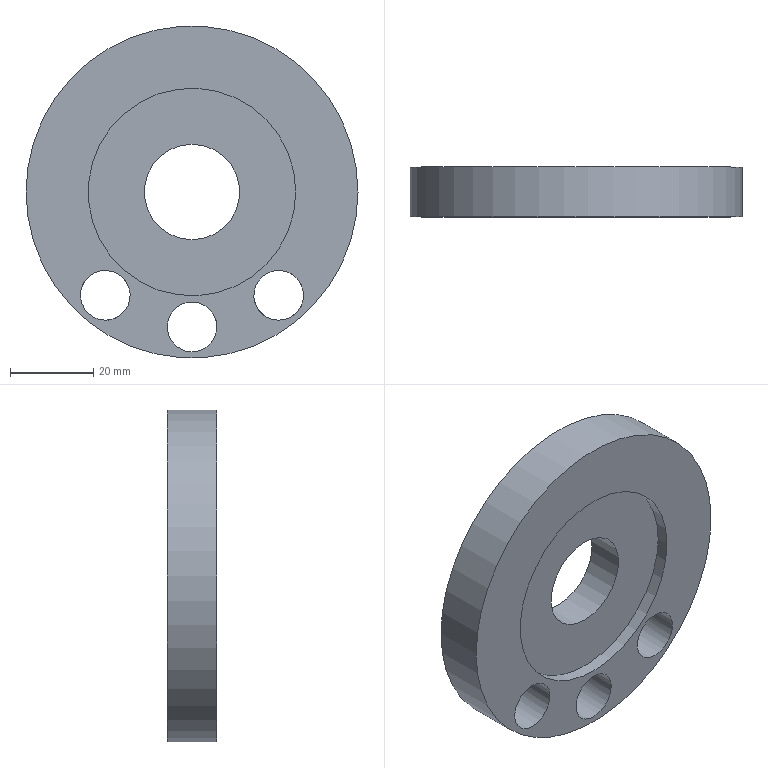Component | NX | INDEXING_PLATE | 1 solid | 9 faces | box 80 x 12 x 80 mm | volume 46617 mm3 | cylinder 6 | plane 3 | commonest cylinder face diameters 12 x3 80 x1 50 x1 23 x1
STEP:
#1=CARTESIAN_POINT('',(0.,0.,0.));
#2=DIRECTION('',(0.,0.,1.));
#3=DIRECTION('',(1.,0.,0.));
#4=AXIS2_PLACEMENT_3D('',#1,#2,#3);
#5=CARTESIAN_POINT('',(40.,-12.,66.));
#6=VERTEX_POINT('',#5);
#7=CARTESIAN_POINT('',(0.,-12.,66.));
#8=DIRECTION('',(0.,-1.,0.));
#9=DIRECTION('',(1.,0.,0.));
#10=AXIS2_PLACEMENT_3D('',#7,#8,#9);
#11=CIRCLE('',#10,40.);
#12=CARTESIAN_POINT('',(0.,-12.,66.));
#13=DIRECTION('',(0.,1.,0.));
#14=DIRECTION('',(0.,0.,1.));
#15=AXIS2_PLACEMENT_3D('',#12,#13,#14);
#16=CYLINDRICAL_SURFACE('',#15,40.);
#17=CARTESIAN_POINT('',(7.854,0.));
#18=DIRECTION('',(-1.,0.));
#19=VECTOR('',#18,1.);
#20=LINE('',#17,#19);
#21=(GEOMETRIC_REPRESENTATION_CONTEXT(2)PARAMETRIC_REPRESENTATION_CONTEXT()REPRESENTATION_CONTEXT('',''));
#22=DEFINITIONAL_REPRESENTATION('',(#20),#21);
#23=PCURVE('',#16,#22);
#24=CARTESIAN_POINT('',(0.,-12.,66.));
#25=DIRECTION('',(0.,-1.,0.));
#26=DIRECTION('',(0.,0.,-1.));
#27=AXIS2_PLACEMENT_3D('',#24,#25,#26);
#28=PLANE('',#27);
#29=CARTESIAN_POINT('',(0.,0.));
#30=DIRECTION('',(0.,1.));
#31=AXIS2_PLACEMENT_2D('',#29,#30);
#32=CIRCLE('',#31,40.);
#33=(GEOMETRIC_REPRESENTATION_CONTEXT(2)PARAMETRIC_REPRESENTATION_CONTEXT()REPRESENTATION_CONTEXT('',''));
#34=DEFINITIONAL_REPRESENTATION('',(#32),#33);
#35=PCURVE('',#28,#34);
#36=SURFACE_CURVE('',#11,(#23,#35),.PCURVE_S1.);
#37=EDGE_CURVE('',#6,#6,#36,.T.);
#38=ORIENTED_EDGE('',*,*,#37,.F.);
#39=CARTESIAN_POINT('',(40.,0.,66.));
#40=VERTEX_POINT('',#39);
#41=CARTESIAN_POINT('',(40.,-12.,66.));
#42=CARTESIAN_POINT('',(40.,0.,66.));
#43=B_SPLINE_CURVE_WITH_KNOTS('',1,(#41,#42),.UNSPECIFIED.,.F.,.F.,(2,2),(0.,12.),.PIECEWISE_BEZIER_KNOTS.);
#44=CARTESIAN_POINT('',(7.854,0.));
#45=DIRECTION('',(0.,1.));
#46=VECTOR('',#45,1.);
#47=LINE('',#44,#46);
#48=(GEOMETRIC_REPRESENTATION_CONTEXT(2)PARAMETRIC_REPRESENTATION_CONTEXT()REPRESENTATION_CONTEXT('',''));
#49=DEFINITIONAL_REPRESENTATION('',(#47),#48);
#50=PCURVE('',#16,#49);
#51=CARTESIAN_POINT('',(1.571,0.));
#52=DIRECTION('',(0.,1.));
#53=VECTOR('',#52,1.);
#54=LINE('',#51,#53);
#55=(GEOMETRIC_REPRESENTATION_CONTEXT(2)PARAMETRIC_REPRESENTATION_CONTEXT()REPRESENTATION_CONTEXT('',''));
#56=DEFINITIONAL_REPRESENTATION('',(#54),#55);
#57=PCURVE('',#16,#56);
#58=SEAM_CURVE('',#43,(#50,#57),.PCURVE_S1.);
#59=EDGE_CURVE('',#6,#40,#58,.T.);
#60=ORIENTED_EDGE('',*,*,#59,.T.);
#61=CARTESIAN_POINT('',(0.,0.,66.));
#62=DIRECTION('',(0.,-1.,0.));
#63=DIRECTION('',(1.,0.,0.));
#64=AXIS2_PLACEMENT_3D('',#61,#62,#63);
#65=CIRCLE('',#64,40.);
#66=CARTESIAN_POINT('',(7.854,12.));
#67=DIRECTION('',(-1.,0.));
#68=VECTOR('',#67,1.);
#69=LINE('',#66,#68);
#70=(GEOMETRIC_REPRESENTATION_CONTEXT(2)PARAMETRIC_REPRESENTATION_CONTEXT()REPRESENTATION_CONTEXT('',''));
#71=DEFINITIONAL_REPRESENTATION('',(#69),#70);
#72=PCURVE('',#16,#71);
#73=CARTESIAN_POINT('',(0.,0.,66.));
#74=DIRECTION('',(0.,-1.,0.));
#75=DIRECTION('',(0.,0.,-1.));
#76=AXIS2_PLACEMENT_3D('',#73,#74,#75);
#77=PLANE('',#76);
#78=CARTESIAN_POINT('',(0.,0.));
#79=DIRECTION('',(0.,1.));
#80=AXIS2_PLACEMENT_2D('',#78,#79);
#81=CIRCLE('',#80,40.);
#82=(GEOMETRIC_REPRESENTATION_CONTEXT(2)PARAMETRIC_REPRESENTATION_CONTEXT()REPRESENTATION_CONTEXT('',''));
#83=DEFINITIONAL_REPRESENTATION('',(#81),#82);
#84=PCURVE('',#77,#83);
#85=SURFACE_CURVE('',#65,(#72,#84),.PCURVE_S1.);
#86=EDGE_CURVE('',#40,#40,#85,.T.);
#87=ORIENTED_EDGE('',*,*,#86,.T.);
#88=ORIENTED_EDGE('',*,*,#59,.F.);
#89=EDGE_LOOP('',(#38,#60,#87,#88));
#90=FACE_BOUND('',#89,.T.);
#91=ADVANCED_FACE('',(#90),#16,.T.);
#92=CARTESIAN_POINT('',(26.891,-12.,41.104));
#93=VERTEX_POINT('',#92);
#94=CARTESIAN_POINT('',(20.891,-12.,35.104));
#95=VERTEX_POINT('',#94);
#96=CARTESIAN_POINT('',(20.891,-12.,41.104));
#97=DIRECTION('',(0.,-1.,0.));
#98=DIRECTION('',(1.,0.,0.));
#99=AXIS2_PLACEMENT_3D('',#96,#97,#98);
#100=CIRCLE('',#99,6.);
#101=CARTESIAN_POINT('',(24.896,20.891));
#102=DIRECTION('',(0.,1.));
#103=AXIS2_PLACEMENT_2D('',#101,#102);
#104=CIRCLE('',#103,6.);
#105=(GEOMETRIC_REPRESENTATION_CONTEXT(2)PARAMETRIC_REPRESENTATION_CONTEXT()REPRESENTATION_CONTEXT('',''));
#106=DEFINITIONAL_REPRESENTATION('',(#104),#105);
#107=PCURVE('',#28,#106);
#108=CARTESIAN_POINT('',(20.891,38.,41.104));
#109=DIRECTION('',(0.,-1.,0.));
#110=DIRECTION('',(0.,0.,-1.));
#111=AXIS2_PLACEMENT_3D('',#108,#109,#110);
#112=CYLINDRICAL_SURFACE('',#111,6.);
#113=CARTESIAN_POINT('',(1.571,50.));
#114=DIRECTION('',(1.,0.));
#115=VECTOR('',#114,1.);
#116=LINE('',#113,#115);
#117=(GEOMETRIC_REPRESENTATION_CONTEXT(2)PARAMETRIC_REPRESENTATION_CONTEXT()REPRESENTATION_CONTEXT('',''));
#118=DEFINITIONAL_REPRESENTATION('',(#116),#117);
#119=PCURVE('',#112,#118);
#120=SURFACE_CURVE('',#100,(#107,#119),.PCURVE_S1.);
#121=EDGE_CURVE('',#93,#95,#120,.T.);
#122=ORIENTED_EDGE('',*,*,#121,.F.);
#123=CARTESIAN_POINT('',(20.891,-12.,41.104));
#124=DIRECTION('',(0.,-1.,0.));
#125=DIRECTION('',(1.,0.,0.));
#126=AXIS2_PLACEMENT_3D('',#123,#124,#125);
#127=CIRCLE('',#126,6.);
#128=CARTESIAN_POINT('',(24.896,20.891));
#129=DIRECTION('',(0.,1.));
#130=AXIS2_PLACEMENT_2D('',#128,#129);
#131=CIRCLE('',#130,6.);
#132=(GEOMETRIC_REPRESENTATION_CONTEXT(2)PARAMETRIC_REPRESENTATION_CONTEXT()REPRESENTATION_CONTEXT('',''));
#133=DEFINITIONAL_REPRESENTATION('',(#131),#132);
#134=PCURVE('',#28,#133);
#135=CARTESIAN_POINT('',(-4.712,50.));
#136=DIRECTION('',(1.,0.));
#137=VECTOR('',#136,1.);
#138=LINE('',#135,#137);
#139=(GEOMETRIC_REPRESENTATION_CONTEXT(2)PARAMETRIC_REPRESENTATION_CONTEXT()REPRESENTATION_CONTEXT('',''));
#140=DEFINITIONAL_REPRESENTATION('',(#138),#139);
#141=PCURVE('',#112,#140);
#142=SURFACE_CURVE('',#127,(#134,#141),.PCURVE_S1.);
#143=EDGE_CURVE('',#95,#93,#142,.T.);
#144=ORIENTED_EDGE('',*,*,#143,.F.);
#145=EDGE_LOOP('',(#122,#144));
#146=FACE_BOUND('',#145,.T.);
#147=CARTESIAN_POINT('',(-19.849,-12.,35.195));
#148=VERTEX_POINT('',#147);
#149=CARTESIAN_POINT('',(-20.891,-12.,35.104));
#150=VERTEX_POINT('',#149);
#151=CARTESIAN_POINT('',(-20.891,-12.,41.104));
#152=DIRECTION('',(0.,-1.,0.));
#153=DIRECTION('',(0.1736,0.,-0.9848));
#154=AXIS2_PLACEMENT_3D('',#151,#152,#153);
#155=CIRCLE('',#154,6.);
#156=CARTESIAN_POINT('',(24.896,-20.891));
#157=DIRECTION('',(0.9848,0.1736));
#158=AXIS2_PLACEMENT_2D('',#156,#157);
#159=CIRCLE('',#158,6.);
#160=(GEOMETRIC_REPRESENTATION_CONTEXT(2)PARAMETRIC_REPRESENTATION_CONTEXT()REPRESENTATION_CONTEXT('',''));
#161=DEFINITIONAL_REPRESENTATION('',(#159),#160);
#162=PCURVE('',#28,#161);
#163=CARTESIAN_POINT('',(-20.891,38.,41.104));
#164=DIRECTION('',(0.,-1.,0.));
#165=DIRECTION('',(0.,0.,-1.));
#166=AXIS2_PLACEMENT_3D('',#163,#164,#165);
#167=CYLINDRICAL_SURFACE('',#166,6.);
#168=CARTESIAN_POINT('',(0.1745,50.));
#169=DIRECTION('',(1.,0.));
#170=VECTOR('',#169,1.);
#171=LINE('',#168,#170);
#172=(GEOMETRIC_REPRESENTATION_CONTEXT(2)PARAMETRIC_REPRESENTATION_CONTEXT()REPRESENTATION_CONTEXT('',''));
#173=DEFINITIONAL_REPRESENTATION('',(#171),#172);
#174=PCURVE('',#167,#173);
#175=SURFACE_CURVE('',#155,(#162,#174),.PCURVE_S1.);
#176=EDGE_CURVE('',#148,#150,#175,.T.);
#177=ORIENTED_EDGE('',*,*,#176,.F.);
#178=CARTESIAN_POINT('',(-20.891,-12.,41.104));
#179=DIRECTION('',(0.,-1.,0.));
#180=DIRECTION('',(0.1736,0.,-0.9848));
#181=AXIS2_PLACEMENT_3D('',#178,#179,#180);
#182=CIRCLE('',#181,6.);
#183=CARTESIAN_POINT('',(24.896,-20.891));
#184=DIRECTION('',(0.9848,0.1736));
#185=AXIS2_PLACEMENT_2D('',#183,#184);
#186=CIRCLE('',#185,6.);
#187=(GEOMETRIC_REPRESENTATION_CONTEXT(2)PARAMETRIC_REPRESENTATION_CONTEXT()REPRESENTATION_CONTEXT('',''));
#188=DEFINITIONAL_REPRESENTATION('',(#186),#187);
#189=PCURVE('',#28,#188);
#190=CARTESIAN_POINT('',(-6.109,50.));
#191=DIRECTION('',(1.,0.));
#192=VECTOR('',#191,1.);
#193=LINE('',#190,#192);
#194=(GEOMETRIC_REPRESENTATION_CONTEXT(2)PARAMETRIC_REPRESENTATION_CONTEXT()REPRESENTATION_CONTEXT('',''));
#195=DEFINITIONAL_REPRESENTATION('',(#193),#194);
#196=PCURVE('',#167,#195);
#197=SURFACE_CURVE('',#182,(#189,#196),.PCURVE_S1.);
#198=EDGE_CURVE('',#150,#148,#197,.T.);
#199=ORIENTED_EDGE('',*,*,#198,.F.);
#200=EDGE_LOOP('',(#177,#199));
#201=FACE_BOUND('',#200,.T.);
#202=CARTESIAN_POINT('',(4.596,-12.,29.643));
#203=VERTEX_POINT('',#202);
#204=CARTESIAN_POINT('',(0.,-12.,27.5));
#205=VERTEX_POINT('',#204);
#206=CARTESIAN_POINT('',(0.,-12.,33.5));
#207=DIRECTION('',(0.,-1.,0.));
#208=DIRECTION('',(0.766,0.,-0.6428));
#209=AXIS2_PLACEMENT_3D('',#206,#207,#208);
#210=CIRCLE('',#209,6.);
#211=CARTESIAN_POINT('',(32.5,0.));
#212=DIRECTION('',(0.6428,0.766));
#213=AXIS2_PLACEMENT_2D('',#211,#212);
#214=CIRCLE('',#213,6.);
#215=(GEOMETRIC_REPRESENTATION_CONTEXT(2)PARAMETRIC_REPRESENTATION_CONTEXT()REPRESENTATION_CONTEXT('',''));
#216=DEFINITIONAL_REPRESENTATION('',(#214),#215);
#217=PCURVE('',#28,#216);
#218=CARTESIAN_POINT('',(0.,38.,33.5));
#219=DIRECTION('',(0.,-1.,0.));
#220=DIRECTION('',(0.,0.,-1.));
#221=AXIS2_PLACEMENT_3D('',#218,#219,#220);
#222=CYLINDRICAL_SURFACE('',#221,6.);
#223=CARTESIAN_POINT('',(0.8727,50.));
#224=DIRECTION('',(1.,0.));
#225=VECTOR('',#224,1.);
#226=LINE('',#223,#225);
#227=(GEOMETRIC_REPRESENTATION_CONTEXT(2)PARAMETRIC_REPRESENTATION_CONTEXT()REPRESENTATION_CONTEXT('',''));
#228=DEFINITIONAL_REPRESENTATION('',(#226),#227);
#229=PCURVE('',#222,#228);
#230=SURFACE_CURVE('',#210,(#217,#229),.PCURVE_S1.);
#231=EDGE_CURVE('',#203,#205,#230,.T.);
#232=ORIENTED_EDGE('',*,*,#231,.F.);
#233=CARTESIAN_POINT('',(0.,-12.,33.5));
#234=DIRECTION('',(0.,-1.,0.));
#235=DIRECTION('',(0.766,0.,-0.6428));
#236=AXIS2_PLACEMENT_3D('',#233,#234,#235);
#237=CIRCLE('',#236,6.);
#238=CARTESIAN_POINT('',(32.5,0.));
#239=DIRECTION('',(0.6428,0.766));
#240=AXIS2_PLACEMENT_2D('',#238,#239);
#241=CIRCLE('',#240,6.);
#242=(GEOMETRIC_REPRESENTATION_CONTEXT(2)PARAMETRIC_REPRESENTATION_CONTEXT()REPRESENTATION_CONTEXT('',''));
#243=DEFINITIONAL_REPRESENTATION('',(#241),#242);
#244=PCURVE('',#28,#243);
#245=CARTESIAN_POINT('',(-5.411,50.));
#246=DIRECTION('',(1.,0.));
#247=VECTOR('',#246,1.);
#248=LINE('',#245,#247);
#249=(GEOMETRIC_REPRESENTATION_CONTEXT(2)PARAMETRIC_REPRESENTATION_CONTEXT()REPRESENTATION_CONTEXT('',''));
#250=DEFINITIONAL_REPRESENTATION('',(#248),#249);
#251=PCURVE('',#222,#250);
#252=SURFACE_CURVE('',#237,(#244,#251),.PCURVE_S1.);
#253=EDGE_CURVE('',#205,#203,#252,.T.);
#254=ORIENTED_EDGE('',*,*,#253,.F.);
#255=EDGE_LOOP('',(#232,#254));
#256=FACE_BOUND('',#255,.T.);
#257=CARTESIAN_POINT('',(25.,-12.,66.));
#258=VERTEX_POINT('',#257);
#259=CARTESIAN_POINT('',(0.,-12.,66.));
#260=DIRECTION('',(0.,-1.,0.));
#261=DIRECTION('',(1.,0.,0.));
#262=AXIS2_PLACEMENT_3D('',#259,#260,#261);
#263=CIRCLE('',#262,25.);
#264=CARTESIAN_POINT('',(0.,0.));
#265=DIRECTION('',(0.,1.));
#266=AXIS2_PLACEMENT_2D('',#264,#265);
#267=CIRCLE('',#266,25.);
#268=(GEOMETRIC_REPRESENTATION_CONTEXT(2)PARAMETRIC_REPRESENTATION_CONTEXT()REPRESENTATION_CONTEXT('',''));
#269=DEFINITIONAL_REPRESENTATION('',(#267),#268);
#270=PCURVE('',#28,#269);
#271=CARTESIAN_POINT('',(0.,-9.,66.));
#272=DIRECTION('',(0.,-1.,0.));
#273=DIRECTION('',(0.,0.,-1.));
#274=AXIS2_PLACEMENT_3D('',#271,#272,#273);
#275=CYLINDRICAL_SURFACE('',#274,25.);
#276=CARTESIAN_POINT('',(1.571,3.));
#277=DIRECTION('',(1.,0.));
#278=VECTOR('',#277,1.);
#279=LINE('',#276,#278);
#280=(GEOMETRIC_REPRESENTATION_CONTEXT(2)PARAMETRIC_REPRESENTATION_CONTEXT()REPRESENTATION_CONTEXT('',''));
#281=DEFINITIONAL_REPRESENTATION('',(#279),#280);
#282=PCURVE('',#275,#281);
#283=SURFACE_CURVE('',#263,(#270,#282),.PCURVE_S1.);
#284=EDGE_CURVE('',#258,#258,#283,.T.);
#285=ORIENTED_EDGE('',*,*,#284,.F.);
#286=EDGE_LOOP('',(#285));
#287=FACE_BOUND('',#286,.T.);
#288=ORIENTED_EDGE('',*,*,#37,.T.);
#289=EDGE_LOOP('',(#288));
#290=FACE_BOUND('',#289,.T.);
#291=ADVANCED_FACE('',(#146,#201,#256,#287,#290),#28,.T.);
#292=CARTESIAN_POINT('',(20.891,0.,35.104));
#293=VERTEX_POINT('',#292);
#294=CARTESIAN_POINT('',(20.891,0.,41.104));
#295=DIRECTION('',(0.,-1.,0.));
#296=DIRECTION('',(0.,0.,-1.));
#297=AXIS2_PLACEMENT_3D('',#294,#295,#296);
#298=CIRCLE('',#297,6.);
#299=CARTESIAN_POINT('',(24.896,20.891));
#300=DIRECTION('',(1.,0.));
#301=AXIS2_PLACEMENT_2D('',#299,#300);
#302=CIRCLE('',#301,6.);
#303=(GEOMETRIC_REPRESENTATION_CONTEXT(2)PARAMETRIC_REPRESENTATION_CONTEXT()REPRESENTATION_CONTEXT('',''));
#304=DEFINITIONAL_REPRESENTATION('',(#302),#303);
#305=PCURVE('',#77,#304);
#306=CARTESIAN_POINT('',(0.,38.));
#307=DIRECTION('',(1.,0.));
#308=VECTOR('',#307,1.);
#309=LINE('',#306,#308);
#310=(GEOMETRIC_REPRESENTATION_CONTEXT(2)PARAMETRIC_REPRESENTATION_CONTEXT()REPRESENTATION_CONTEXT('',''));
#311=DEFINITIONAL_REPRESENTATION('',(#309),#310);
#312=PCURVE('',#112,#311);
#313=SURFACE_CURVE('',#298,(#305,#312),.PCURVE_S1.);
#314=EDGE_CURVE('',#293,#293,#313,.T.);
#315=ORIENTED_EDGE('',*,*,#314,.T.);
#316=EDGE_LOOP('',(#315));
#317=FACE_BOUND('',#316,.T.);
#318=CARTESIAN_POINT('',(-20.891,0.,35.104));
#319=VERTEX_POINT('',#318);
#320=CARTESIAN_POINT('',(-20.891,0.,41.104));
#321=DIRECTION('',(0.,-1.,0.));
#322=DIRECTION('',(0.,0.,-1.));
#323=AXIS2_PLACEMENT_3D('',#320,#321,#322);
#324=CIRCLE('',#323,6.);
#325=CARTESIAN_POINT('',(24.896,-20.891));
#326=DIRECTION('',(1.,0.));
#327=AXIS2_PLACEMENT_2D('',#325,#326);
#328=CIRCLE('',#327,6.);
#329=(GEOMETRIC_REPRESENTATION_CONTEXT(2)PARAMETRIC_REPRESENTATION_CONTEXT()REPRESENTATION_CONTEXT('',''));
#330=DEFINITIONAL_REPRESENTATION('',(#328),#329);
#331=PCURVE('',#77,#330);
#332=CARTESIAN_POINT('',(0.,38.));
#333=DIRECTION('',(1.,0.));
#334=VECTOR('',#333,1.);
#335=LINE('',#332,#334);
#336=(GEOMETRIC_REPRESENTATION_CONTEXT(2)PARAMETRIC_REPRESENTATION_CONTEXT()REPRESENTATION_CONTEXT('',''));
#337=DEFINITIONAL_REPRESENTATION('',(#335),#336);
#338=PCURVE('',#167,#337);
#339=SURFACE_CURVE('',#324,(#331,#338),.PCURVE_S1.);
#340=EDGE_CURVE('',#319,#319,#339,.T.);
#341=ORIENTED_EDGE('',*,*,#340,.T.);
#342=EDGE_LOOP('',(#341));
#343=FACE_BOUND('',#342,.T.);
#344=CARTESIAN_POINT('',(0.,0.,27.5));
#345=VERTEX_POINT('',#344);
#346=CARTESIAN_POINT('',(0.,0.,33.5));
#347=DIRECTION('',(0.,-1.,0.));
#348=DIRECTION('',(0.,0.,-1.));
#349=AXIS2_PLACEMENT_3D('',#346,#347,#348);
#350=CIRCLE('',#349,6.);
#351=CARTESIAN_POINT('',(32.5,0.));
#352=DIRECTION('',(1.,0.));
#353=AXIS2_PLACEMENT_2D('',#351,#352);
#354=CIRCLE('',#353,6.);
#355=(GEOMETRIC_REPRESENTATION_CONTEXT(2)PARAMETRIC_REPRESENTATION_CONTEXT()REPRESENTATION_CONTEXT('',''));
#356=DEFINITIONAL_REPRESENTATION('',(#354),#355);
#357=PCURVE('',#77,#356);
#358=CARTESIAN_POINT('',(0.,38.));
#359=DIRECTION('',(1.,0.));
#360=VECTOR('',#359,1.);
#361=LINE('',#358,#360);
#362=(GEOMETRIC_REPRESENTATION_CONTEXT(2)PARAMETRIC_REPRESENTATION_CONTEXT()REPRESENTATION_CONTEXT('',''));
#363=DEFINITIONAL_REPRESENTATION('',(#361),#362);
#364=PCURVE('',#222,#363);
#365=SURFACE_CURVE('',#350,(#357,#364),.PCURVE_S1.);
#366=EDGE_CURVE('',#345,#345,#365,.T.);
#367=ORIENTED_EDGE('',*,*,#366,.T.);
#368=EDGE_LOOP('',(#367));
#369=FACE_BOUND('',#368,.T.);
#370=CARTESIAN_POINT('',(0.,0.,54.5));
#371=VERTEX_POINT('',#370);
#372=CARTESIAN_POINT('',(0.,0.,77.5));
#373=VERTEX_POINT('',#372);
#374=CARTESIAN_POINT('',(0.,0.,66.));
#375=DIRECTION('',(0.,-1.,0.));
#376=DIRECTION('',(0.,0.,-1.));
#377=AXIS2_PLACEMENT_3D('',#374,#375,#376);
#378=CIRCLE('',#377,11.5);
#379=CARTESIAN_POINT('',(0.,0.));
#380=DIRECTION('',(1.,0.));
#381=AXIS2_PLACEMENT_2D('',#379,#380);
#382=CIRCLE('',#381,11.5);
#383=(GEOMETRIC_REPRESENTATION_CONTEXT(2)PARAMETRIC_REPRESENTATION_CONTEXT()REPRESENTATION_CONTEXT('',''));
#384=DEFINITIONAL_REPRESENTATION('',(#382),#383);
#385=PCURVE('',#77,#384);
#386=CARTESIAN_POINT('',(0.,-9.,66.));
#387=DIRECTION('',(0.,1.,0.));
#388=DIRECTION('',(0.,0.,1.));
#389=AXIS2_PLACEMENT_3D('',#386,#387,#388);
#390=CYLINDRICAL_SURFACE('',#389,11.5);
#391=CARTESIAN_POINT('',(3.142,9.));
#392=DIRECTION('',(-1.,0.));
#393=VECTOR('',#392,1.);
#394=LINE('',#391,#393);
#395=(GEOMETRIC_REPRESENTATION_CONTEXT(2)PARAMETRIC_REPRESENTATION_CONTEXT()REPRESENTATION_CONTEXT('',''));
#396=DEFINITIONAL_REPRESENTATION('',(#394),#395);
#397=PCURVE('',#390,#396);
#398=SURFACE_CURVE('',#378,(#385,#397),.PCURVE_S1.);
#399=EDGE_CURVE('',#371,#373,#398,.T.);
#400=ORIENTED_EDGE('',*,*,#399,.T.);
#401=CARTESIAN_POINT('',(0.,0.,66.));
#402=DIRECTION('',(0.,-1.,0.));
#403=DIRECTION('',(0.,0.,-1.));
#404=AXIS2_PLACEMENT_3D('',#401,#402,#403);
#405=CIRCLE('',#404,11.5);
#406=CARTESIAN_POINT('',(0.,0.));
#407=DIRECTION('',(1.,0.));
#408=AXIS2_PLACEMENT_2D('',#406,#407);
#409=CIRCLE('',#408,11.5);
#410=(GEOMETRIC_REPRESENTATION_CONTEXT(2)PARAMETRIC_REPRESENTATION_CONTEXT()REPRESENTATION_CONTEXT('',''));
#411=DEFINITIONAL_REPRESENTATION('',(#409),#410);
#412=PCURVE('',#77,#411);
#413=CARTESIAN_POINT('',(9.425,9.));
#414=DIRECTION('',(-1.,0.));
#415=VECTOR('',#414,1.);
#416=LINE('',#413,#415);
#417=(GEOMETRIC_REPRESENTATION_CONTEXT(2)PARAMETRIC_REPRESENTATION_CONTEXT()REPRESENTATION_CONTEXT('',''));
#418=DEFINITIONAL_REPRESENTATION('',(#416),#417);
#419=PCURVE('',#390,#418);
#420=SURFACE_CURVE('',#405,(#412,#419),.PCURVE_S1.);
#421=EDGE_CURVE('',#373,#371,#420,.T.);
#422=ORIENTED_EDGE('',*,*,#421,.T.);
#423=EDGE_LOOP('',(#400,#422));
#424=FACE_BOUND('',#423,.T.);
#425=ORIENTED_EDGE('',*,*,#86,.F.);
#426=EDGE_LOOP('',(#425));
#427=FACE_BOUND('',#426,.T.);
#428=ADVANCED_FACE('',(#317,#343,#369,#424,#427),#77,.F.);
#429=CARTESIAN_POINT('',(25.,-9.,66.));
#430=VERTEX_POINT('',#429);
#431=CARTESIAN_POINT('',(0.,-9.,66.));
#432=DIRECTION('',(0.,1.,0.));
#433=DIRECTION('',(1.,0.,0.));
#434=AXIS2_PLACEMENT_3D('',#431,#432,#433);
#435=CIRCLE('',#434,25.);
#436=CARTESIAN_POINT('',(7.854,0.));
#437=DIRECTION('',(-1.,0.));
#438=VECTOR('',#437,1.);
#439=LINE('',#436,#438);
#440=(GEOMETRIC_REPRESENTATION_CONTEXT(2)PARAMETRIC_REPRESENTATION_CONTEXT()REPRESENTATION_CONTEXT('',''));
#441=DEFINITIONAL_REPRESENTATION('',(#439),#440);
#442=PCURVE('',#275,#441);
#443=CARTESIAN_POINT('',(0.,-9.,66.));
#444=DIRECTION('',(0.,-1.,0.));
#445=DIRECTION('',(0.,0.,-1.));
#446=AXIS2_PLACEMENT_3D('',#443,#444,#445);
#447=PLANE('',#446);
#448=CARTESIAN_POINT('',(0.,25.));
#449=CARTESIAN_POINT('',(43.301,25.));
#450=CARTESIAN_POINT('',(21.651,-12.5));
#451=CARTESIAN_POINT('',(0.,-50.));
#452=CARTESIAN_POINT('',(-21.651,-12.5));
#453=CARTESIAN_POINT('',(-43.301,25.));
#454=CARTESIAN_POINT('',(0.,25.));
#455=(BOUNDED_CURVE()B_SPLINE_CURVE(2,(#448,#449,#450,#451,#452,#453,#454),.UNSPECIFIED.,.T.,.F.)B_SPLINE_CURVE_WITH_KNOTS((1,2,2,2,2,1),(-2.094,0.,2.094,4.189,6.283,8.378),.UNSPECIFIED.)CURVE()GEOMETRIC_REPRESENTATION_ITEM()RATIONAL_B_SPLINE_CURVE((1.,0.5,1.,0.5,1.,0.5,1.))REPRESENTATION_ITEM(''));
#456=(GEOMETRIC_REPRESENTATION_CONTEXT(2)PARAMETRIC_REPRESENTATION_CONTEXT()REPRESENTATION_CONTEXT('',''));
#457=DEFINITIONAL_REPRESENTATION('',(#455),#456);
#458=PCURVE('',#447,#457);
#459=SURFACE_CURVE('',#435,(#442,#458),.PCURVE_S1.);
#460=EDGE_CURVE('',#430,#430,#459,.T.);
#461=ORIENTED_EDGE('',*,*,#460,.F.);
#462=CARTESIAN_POINT('',(25.,-9.,66.));
#463=CARTESIAN_POINT('',(25.,-12.,66.));
#464=B_SPLINE_CURVE_WITH_KNOTS('',1,(#462,#463),.UNSPECIFIED.,.F.,.F.,(2,2),(0.,3.),.PIECEWISE_BEZIER_KNOTS.);
#465=CARTESIAN_POINT('',(7.854,0.));
#466=DIRECTION('',(0.,1.));
#467=VECTOR('',#466,1.);
#468=LINE('',#465,#467);
#469=(GEOMETRIC_REPRESENTATION_CONTEXT(2)PARAMETRIC_REPRESENTATION_CONTEXT()REPRESENTATION_CONTEXT('',''));
#470=DEFINITIONAL_REPRESENTATION('',(#468),#469);
#471=PCURVE('',#275,#470);
#472=CARTESIAN_POINT('',(1.571,0.));
#473=DIRECTION('',(0.,1.));
#474=VECTOR('',#473,1.);
#475=LINE('',#472,#474);
#476=(GEOMETRIC_REPRESENTATION_CONTEXT(2)PARAMETRIC_REPRESENTATION_CONTEXT()REPRESENTATION_CONTEXT('',''));
#477=DEFINITIONAL_REPRESENTATION('',(#475),#476);
#478=PCURVE('',#275,#477);
#479=SEAM_CURVE('',#464,(#471,#478),.PCURVE_S1.);
#480=EDGE_CURVE('',#430,#258,#479,.T.);
#481=ORIENTED_EDGE('',*,*,#480,.T.);
#482=ORIENTED_EDGE('',*,*,#284,.F.);
#483=ORIENTED_EDGE('',*,*,#480,.F.);
#484=EDGE_LOOP('',(#461,#481,#482,#483));
#485=FACE_BOUND('',#484,.F.);
#486=ADVANCED_FACE('',(#485),#275,.F.);
#487=CARTESIAN_POINT('',(0.,-9.,77.5));
#488=VERTEX_POINT('',#487);
#489=CARTESIAN_POINT('',(0.,-9.,66.));
#490=DIRECTION('',(0.,1.,0.));
#491=DIRECTION('',(0.,0.,1.));
#492=AXIS2_PLACEMENT_3D('',#489,#490,#491);
#493=CIRCLE('',#492,11.5);
#494=CARTESIAN_POINT('',(-11.5,0.));
#495=CARTESIAN_POINT('',(-11.5,19.919));
#496=CARTESIAN_POINT('',(5.75,9.959));
#497=CARTESIAN_POINT('',(23.,0.));
#498=CARTESIAN_POINT('',(5.75,-9.959));
#499=CARTESIAN_POINT('',(-11.5,-19.919));
#500=CARTESIAN_POINT('',(-11.5,0.));
#501=(BOUNDED_CURVE()B_SPLINE_CURVE(2,(#494,#495,#496,#497,#498,#499,#500),.UNSPECIFIED.,.T.,.F.)B_SPLINE_CURVE_WITH_KNOTS((1,2,2,2,2,1),(-2.094,0.,2.094,4.189,6.283,8.378),.UNSPECIFIED.)CURVE()GEOMETRIC_REPRESENTATION_ITEM()RATIONAL_B_SPLINE_CURVE((1.,0.5,1.,0.5,1.,0.5,1.))REPRESENTATION_ITEM(''));
#502=(GEOMETRIC_REPRESENTATION_CONTEXT(2)PARAMETRIC_REPRESENTATION_CONTEXT()REPRESENTATION_CONTEXT('',''));
#503=DEFINITIONAL_REPRESENTATION('',(#501),#502);
#504=PCURVE('',#447,#503);
#505=CARTESIAN_POINT('',(0.,0.));
#506=DIRECTION('',(1.,0.));
#507=VECTOR('',#506,1.);
#508=LINE('',#505,#507);
#509=(GEOMETRIC_REPRESENTATION_CONTEXT(2)PARAMETRIC_REPRESENTATION_CONTEXT()REPRESENTATION_CONTEXT('',''));
#510=DEFINITIONAL_REPRESENTATION('',(#508),#509);
#511=PCURVE('',#390,#510);
#512=SURFACE_CURVE('',#493,(#504,#511),.PCURVE_S1.);
#513=EDGE_CURVE('',#488,#488,#512,.T.);
#514=ORIENTED_EDGE('',*,*,#513,.T.);
#515=EDGE_LOOP('',(#514));
#516=FACE_BOUND('',#515,.T.);
#517=ORIENTED_EDGE('',*,*,#460,.F.);
#518=EDGE_LOOP('',(#517));
#519=FACE_BOUND('',#518,.T.);
#520=ADVANCED_FACE('',(#516,#519),#447,.T.);
#521=ORIENTED_EDGE('',*,*,#513,.T.);
#522=CARTESIAN_POINT('',(0.,-9.,77.5));
#523=CARTESIAN_POINT('',(0.,0.,77.5));
#524=B_SPLINE_CURVE_WITH_KNOTS('',1,(#522,#523),.UNSPECIFIED.,.F.,.F.,(2,2),(0.,9.),.PIECEWISE_BEZIER_KNOTS.);
#525=CARTESIAN_POINT('',(6.283,0.));
#526=DIRECTION('',(0.,1.));
#527=VECTOR('',#526,1.);
#528=LINE('',#525,#527);
#529=(GEOMETRIC_REPRESENTATION_CONTEXT(2)PARAMETRIC_REPRESENTATION_CONTEXT()REPRESENTATION_CONTEXT('',''));
#530=DEFINITIONAL_REPRESENTATION('',(#528),#529);
#531=PCURVE('',#390,#530);
#532=CARTESIAN_POINT('',(0.,0.));
#533=DIRECTION('',(0.,1.));
#534=VECTOR('',#533,1.);
#535=LINE('',#532,#534);
#536=(GEOMETRIC_REPRESENTATION_CONTEXT(2)PARAMETRIC_REPRESENTATION_CONTEXT()REPRESENTATION_CONTEXT('',''));
#537=DEFINITIONAL_REPRESENTATION('',(#535),#536);
#538=PCURVE('',#390,#537);
#539=SEAM_CURVE('',#524,(#531,#538),.PCURVE_S1.);
#540=EDGE_CURVE('',#488,#373,#539,.T.);
#541=ORIENTED_EDGE('',*,*,#540,.T.);
#542=ORIENTED_EDGE('',*,*,#421,.T.);
#543=ORIENTED_EDGE('',*,*,#399,.T.);
#544=ORIENTED_EDGE('',*,*,#540,.F.);
#545=EDGE_LOOP('',(#521,#541,#542,#543,#544));
#546=FACE_BOUND('',#545,.F.);
#547=ADVANCED_FACE('',(#546),#390,.F.);
#548=ORIENTED_EDGE('',*,*,#253,.F.);
#549=CARTESIAN_POINT('',(0.,0.,27.5));
#550=CARTESIAN_POINT('',(0.,-12.,27.5));
#551=B_SPLINE_CURVE_WITH_KNOTS('',1,(#549,#550),.UNSPECIFIED.,.F.,.F.,(2,2),(38.,50.),.PIECEWISE_BEZIER_KNOTS.);
#552=CARTESIAN_POINT('',(0.,0.));
#553=DIRECTION('',(0.,1.));
#554=VECTOR('',#553,1.);
#555=LINE('',#552,#554);
#556=(GEOMETRIC_REPRESENTATION_CONTEXT(2)PARAMETRIC_REPRESENTATION_CONTEXT()REPRESENTATION_CONTEXT('',''));
#557=DEFINITIONAL_REPRESENTATION('',(#555),#556);
#558=PCURVE('',#222,#557);
#559=CARTESIAN_POINT('',(6.283,0.));
#560=DIRECTION('',(0.,1.));
#561=VECTOR('',#560,1.);
#562=LINE('',#559,#561);
#563=(GEOMETRIC_REPRESENTATION_CONTEXT(2)PARAMETRIC_REPRESENTATION_CONTEXT()REPRESENTATION_CONTEXT('',''));
#564=DEFINITIONAL_REPRESENTATION('',(#562),#563);
#565=PCURVE('',#222,#564);
#566=SEAM_CURVE('',#551,(#558,#565),.PCURVE_S1.);
#567=EDGE_CURVE('',#345,#205,#566,.T.);
#568=ORIENTED_EDGE('',*,*,#567,.F.);
#569=ORIENTED_EDGE('',*,*,#366,.T.);
#570=ORIENTED_EDGE('',*,*,#567,.T.);
#571=ORIENTED_EDGE('',*,*,#231,.F.);
#572=EDGE_LOOP('',(#548,#568,#569,#570,#571));
#573=FACE_BOUND('',#572,.F.);
#574=ADVANCED_FACE('',(#573),#222,.F.);
#575=ORIENTED_EDGE('',*,*,#198,.F.);
#576=CARTESIAN_POINT('',(-20.891,0.,35.104));
#577=CARTESIAN_POINT('',(-20.891,-12.,35.104));
#578=B_SPLINE_CURVE_WITH_KNOTS('',1,(#576,#577),.UNSPECIFIED.,.F.,.F.,(2,2),(38.,50.),.PIECEWISE_BEZIER_KNOTS.);
#579=CARTESIAN_POINT('',(0.,0.));
#580=DIRECTION('',(0.,1.));
#581=VECTOR('',#580,1.);
#582=LINE('',#579,#581);
#583=(GEOMETRIC_REPRESENTATION_CONTEXT(2)PARAMETRIC_REPRESENTATION_CONTEXT()REPRESENTATION_CONTEXT('',''));
#584=DEFINITIONAL_REPRESENTATION('',(#582),#583);
#585=PCURVE('',#167,#584);
#586=CARTESIAN_POINT('',(6.283,0.));
#587=DIRECTION('',(0.,1.));
#588=VECTOR('',#587,1.);
#589=LINE('',#586,#588);
#590=(GEOMETRIC_REPRESENTATION_CONTEXT(2)PARAMETRIC_REPRESENTATION_CONTEXT()REPRESENTATION_CONTEXT('',''));
#591=DEFINITIONAL_REPRESENTATION('',(#589),#590);
#592=PCURVE('',#167,#591);
#593=SEAM_CURVE('',#578,(#585,#592),.PCURVE_S1.);
#594=EDGE_CURVE('',#319,#150,#593,.T.);
#595=ORIENTED_EDGE('',*,*,#594,.F.);
#596=ORIENTED_EDGE('',*,*,#340,.T.);
#597=ORIENTED_EDGE('',*,*,#594,.T.);
#598=ORIENTED_EDGE('',*,*,#176,.F.);
#599=EDGE_LOOP('',(#575,#595,#596,#597,#598));
#600=FACE_BOUND('',#599,.F.);
#601=ADVANCED_FACE('',(#600),#167,.F.);
#602=ORIENTED_EDGE('',*,*,#143,.F.);
#603=CARTESIAN_POINT('',(20.891,0.,35.104));
#604=CARTESIAN_POINT('',(20.891,-12.,35.104));
#605=B_SPLINE_CURVE_WITH_KNOTS('',1,(#603,#604),.UNSPECIFIED.,.F.,.F.,(2,2),(38.,50.),.PIECEWISE_BEZIER_KNOTS.);
#606=CARTESIAN_POINT('',(0.,0.));
#607=DIRECTION('',(0.,1.));
#608=VECTOR('',#607,1.);
#609=LINE('',#606,#608);
#610=(GEOMETRIC_REPRESENTATION_CONTEXT(2)PARAMETRIC_REPRESENTATION_CONTEXT()REPRESENTATION_CONTEXT('',''));
#611=DEFINITIONAL_REPRESENTATION('',(#609),#610);
#612=PCURVE('',#112,#611);
#613=CARTESIAN_POINT('',(6.283,0.));
#614=DIRECTION('',(0.,1.));
#615=VECTOR('',#614,1.);
#616=LINE('',#613,#615);
#617=(GEOMETRIC_REPRESENTATION_CONTEXT(2)PARAMETRIC_REPRESENTATION_CONTEXT()REPRESENTATION_CONTEXT('',''));
#618=DEFINITIONAL_REPRESENTATION('',(#616),#617);
#619=PCURVE('',#112,#618);
#620=SEAM_CURVE('',#605,(#612,#619),.PCURVE_S1.);
#621=EDGE_CURVE('',#293,#95,#620,.T.);
#622=ORIENTED_EDGE('',*,*,#621,.F.);
#623=ORIENTED_EDGE('',*,*,#314,.T.);
#624=ORIENTED_EDGE('',*,*,#621,.T.);
#625=ORIENTED_EDGE('',*,*,#121,.F.);
#626=EDGE_LOOP('',(#602,#622,#623,#624,#625));
#627=FACE_BOUND('',#626,.F.);
#628=ADVANCED_FACE('',(#627),#112,.F.);
#629=CLOSED_SHELL('',(#91,#291,#428,#486,#520,#547,#574,#601,#628));
#630=MANIFOLD_SOLID_BREP('',#629);
#631=(LENGTH_UNIT()NAMED_UNIT(*)SI_UNIT(.MILLI.,.METRE.));
#632=UNCERTAINTY_MEASURE_WITH_UNIT(LENGTH_MEASURE(0.000005),#631,'','');
#633=(NAMED_UNIT(*)PLANE_ANGLE_UNIT()SI_UNIT($,.RADIAN.));
#634=(NAMED_UNIT(*)SI_UNIT($,.STERADIAN.)SOLID_ANGLE_UNIT());
#635=(GEOMETRIC_REPRESENTATION_CONTEXT(3)GLOBAL_UNCERTAINTY_ASSIGNED_CONTEXT((#632))GLOBAL_UNIT_ASSIGNED_CONTEXT((#631,#633,#634))REPRESENTATION_CONTEXT('',''));
#636=ADVANCED_BREP_SHAPE_REPRESENTATION('',(#4,#630),#635);